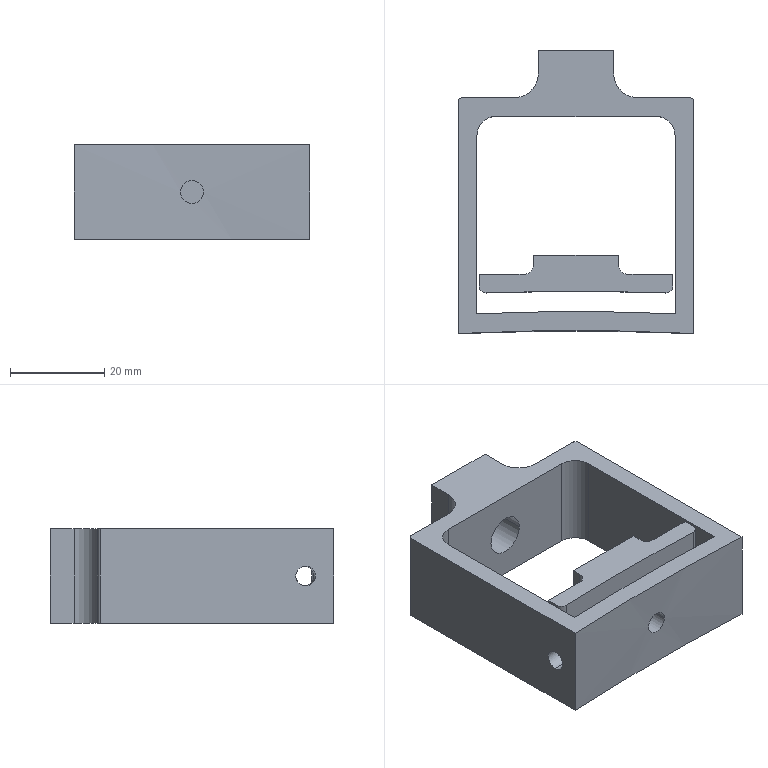CAM job | Mastercam | mm | 8 operations | part box 50 x 60 x 20
1. Contour (Ramp) | 6 - 6 平铣刀
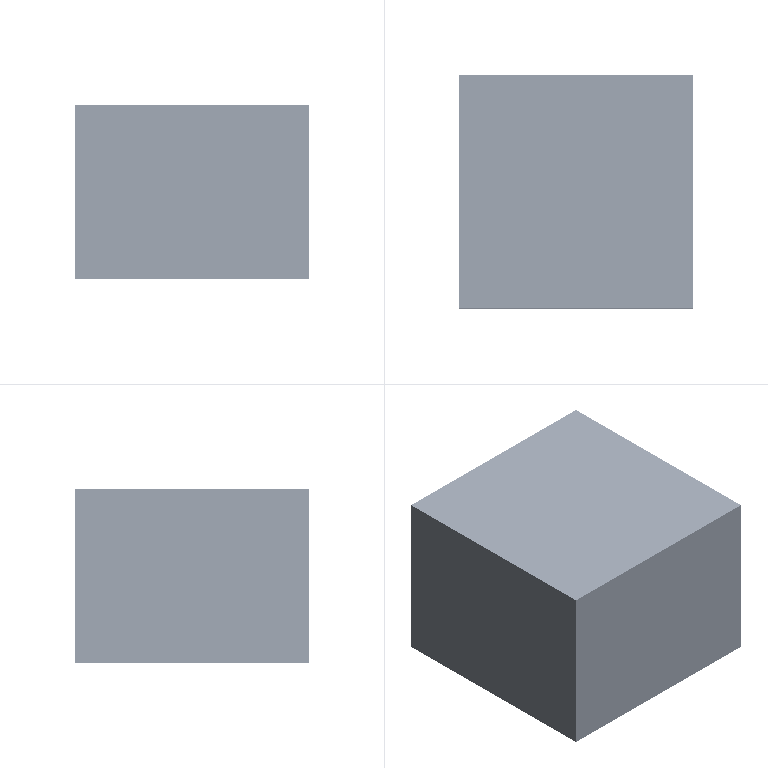2. Contour (2D) | 6 - 6 平铣刀
3. Contour (Ramp) | 6 - 6 平铣刀
4. Contour (2D) | 6 - 6 平铣刀
5. Contour (2D chamfer) | 7 - 4 倒角刀
6. Contour (Ramp) | 6 - 6 平铣刀
7. Contour (2D chamfer) | 7 - 4 倒角刀
8. Drill/Counterbore | 7 - 4 倒角刀